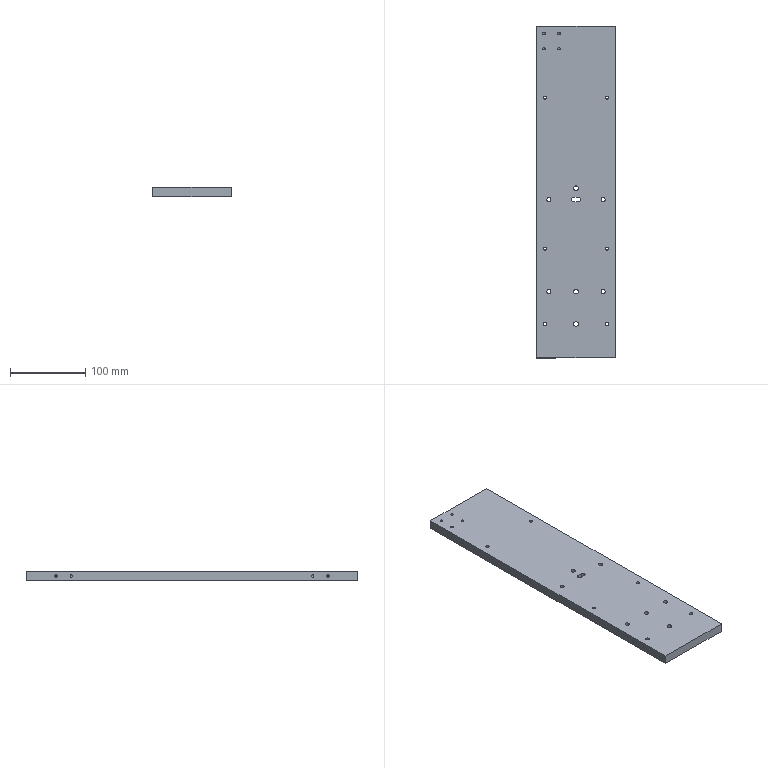Component | SolidWorks | 005-1 | 1 solid | 101 faces | box 105 x 440 x 12 mm | volume 548147 mm3 | cylinder 61 | cone 24 | plane 16 | commonest cylinder face diameters 3.3 x24 4.2 x12 6 x9 10 x8 5.5 x8 | material AL6061
build123d program:
from build123d import *

# Parameters (mm, degrees)
SKETCH1_W                                         = 105
SKETCH1_H                                         = 440
BOSS_EXTRUDE1_DEPTH                               = 12
CHAMFER1_SIZE                                     = 0.5
HOLE_SIZE_ACCORDING_TO_TYPE_OF_HEX_SO_D           = 5.5
HOLE_SIZE_ACCORDING_TO_TYPE_OF_HEX_SO_DEPTH       = 15
HOLE_SIZE_ACCORDING_TO_TYPE_OF_HEX_SO_CBORE_D     = 10
HOLE_SIZE_ACCORDING_TO_TYPE_OF_HEX_SO_CBORE_DEPTH = 5.7
HOLE_SIZE_ACCORDING_TO_TYPE_OF_HEX_SO_TIP         = 1.652
SKETCH4_R                                         = 3
CUT_EXTRUDE1_DEPTH                                = 227.496
M5_TAPPED_HOLE1_D                                 = 4.2
M5_TAPPED_HOLE1_DEPTH                             = 12.4
M5_TAPPED_HOLE1_TIP                               = 1.262
SIZE_MM_DOWEL_PIN_HOLE1_D                         = 6
SIZE_MM_DOWEL_PIN_HOLE1_DEPTH                     = 12.4
SIZE_MM_DOWEL_PIN_HOLE1_TIP                       = 1.803
M4_TAPPED_HOLE1_D                                 = 3.3
M4_TAPPED_HOLE1_DEPTH                             = 10.1
M4_TAPPED_HOLE1_TIP                               = 0.9914
M4_TAPPED_HOLE2_AT_2_COUNT                        = 2
M4_TAPPED_HOLE2_AT_2_PITCH                        = 20
M4_TAPPED_HOLE2_AT_3_COUNT                        = 2
M4_TAPPED_HOLE2_AT_3_PITCH                        = 360
M4_TAPPED_HOLE2_AT_4_COUNT                        = 2
M4_TAPPED_HOLE2_AT_4_PITCH                        = 340


with BuildPart() as part:
    # Sketch1 → Boss-Extrude1 (new body)
    with BuildSketch(Plane.XY):
        Rectangle(SKETCH1_W, SKETCH1_H)
    extrude(amount=BOSS_EXTRUDE1_DEPTH)

    # Chamfer1
    chamfer1_edges = [part.edges().sort_by_distance(p)[0] for p in [
        (52.5, -220, 6),
        (-52.5, -220, 6),
        (-52.5, 220, 6),
        (52.5, 220, 6),
    ]]
    chamfer(chamfer1_edges, length=CHAMFER1_SIZE)

    # Hole Size _ according to_ type of hex so
    with Locations(Plane.XY.offset(12)):
        with Locations((-36, -10), (36, -132), (-36, -132), (36, -10)):
            CounterBoreHole(HOLE_SIZE_ACCORDING_TO_TYPE_OF_HEX_SO_D / 2, HOLE_SIZE_ACCORDING_TO_TYPE_OF_HEX_SO_CBORE_D / 2, HOLE_SIZE_ACCORDING_TO_TYPE_OF_HEX_SO_CBORE_DEPTH, depth=HOLE_SIZE_ACCORDING_TO_TYPE_OF_HEX_SO_DEPTH)
            with Locations((0, 0, -(HOLE_SIZE_ACCORDING_TO_TYPE_OF_HEX_SO_DEPTH + HOLE_SIZE_ACCORDING_TO_TYPE_OF_HEX_SO_TIP / 2))):  # 118° drill point
                Cone(0, HOLE_SIZE_ACCORDING_TO_TYPE_OF_HEX_SO_D / 2, HOLE_SIZE_ACCORDING_TO_TYPE_OF_HEX_SO_TIP, mode=Mode.SUBTRACT)

    # Sketch4 → Cut-Extrude1 (cut, through all)
    with BuildSketch(Plane.XY.offset(12)):
        with Locations((0, -132)):
            Circle(SKETCH4_R)
        with BuildLine():
            Line((-3, -7), (3, -7))
            ThreePointArc((3, -7), (6, -10), (3, -13))
            Line((3, -13), (-3, -13))
            ThreePointArc((-3, -13), (-6, -10), (-3, -7))
        make_face()
    extrude(amount=-CUT_EXTRUDE1_DEPTH, mode=Mode.SUBTRACT)

    # M5 Tapped Hole1
    with Locations(Plane.XY.offset(12)):
        with Locations((-41, -175), (41, -75), (-41, -75), (41, -175), (41, 125), (-41, 125)):
            Hole(M5_TAPPED_HOLE1_D / 2, depth=M5_TAPPED_HOLE1_DEPTH)
            with Locations((0, 0, -(M5_TAPPED_HOLE1_DEPTH + M5_TAPPED_HOLE1_TIP / 2))):  # 118° drill point
                Cone(0, M5_TAPPED_HOLE1_D / 2, M5_TAPPED_HOLE1_TIP, mode=Mode.SUBTRACT)

    # Size mm Dowel Pin Hole1
    with Locations(Plane.XY.offset(12)):
        with Locations((0, -175), (0, 5)):
            Hole(SIZE_MM_DOWEL_PIN_HOLE1_D / 2, depth=SIZE_MM_DOWEL_PIN_HOLE1_DEPTH)
            with Locations((0, 0, -(SIZE_MM_DOWEL_PIN_HOLE1_DEPTH + SIZE_MM_DOWEL_PIN_HOLE1_TIP / 2))):  # 118° drill point
                Cone(0, SIZE_MM_DOWEL_PIN_HOLE1_D / 2, SIZE_MM_DOWEL_PIN_HOLE1_TIP, mode=Mode.SUBTRACT)

    # M4 Tapped Hole1
    with Locations(Plane(origin=(0, 0, 0), x_dir=(-1, 0, 0), z_dir=(0, 0, -1))):
        with Locations((-42.5, 210), (-22.5, 190), (-42.5, 190), (-22.5, 210)):
            Hole(M4_TAPPED_HOLE1_D / 2, depth=M4_TAPPED_HOLE1_DEPTH)
            with Locations((0, 0, -(M4_TAPPED_HOLE1_DEPTH + M4_TAPPED_HOLE1_TIP / 2))):  # 118° drill point
                Cone(0, M4_TAPPED_HOLE1_D / 2, M4_TAPPED_HOLE1_TIP, mode=Mode.SUBTRACT)

    # Sketch13 → M4 Tapped Hole2 (revolve, cut)
    with BuildSketch(Plane(origin=(-52.5, 180, 6), x_dir=(0, 0, 1), z_dir=(0, 1, 0))):
        Polygon((0, 0), (0, 11.091), (1.65, 10.1), (1.65, 0), align=None)
    m4_tapped_hole2 = revolve(axis=Axis((-58.85, 180, 6), (1, 0, 0)), mode=Mode.SUBTRACT)

    # M4 Tapped Hole2 at 2: M4 Tapped Hole2 ×2
    with Locations(*[(0, -i * M4_TAPPED_HOLE2_AT_2_PITCH, 0) for i in range(1, M4_TAPPED_HOLE2_AT_2_COUNT)]):
        add(m4_tapped_hole2, mode=Mode.SUBTRACT)

    # M4 Tapped Hole2 at 3: M4 Tapped Hole2 ×2
    with Locations(*[(0, -i * M4_TAPPED_HOLE2_AT_3_PITCH, 0) for i in range(1, M4_TAPPED_HOLE2_AT_3_COUNT)]):
        add(m4_tapped_hole2, mode=Mode.SUBTRACT)

    # M4 Tapped Hole2 at 4: M4 Tapped Hole2 ×2
    with Locations(*[(0, -i * M4_TAPPED_HOLE2_AT_4_PITCH, 0) for i in range(1, M4_TAPPED_HOLE2_AT_4_COUNT)]):
        add(m4_tapped_hole2, mode=Mode.SUBTRACT)

    # Mirror1: M4 Tapped Hole2 across plane
    add(m4_tapped_hole2.mirror(Plane.ZY), mode=Mode.SUBTRACT)

    # Mirror1 copy 1 sketch → Mirror1 copy 1 (revolve, cut)
    with BuildSketch(Plane(origin=(52.5, 160, 6), x_dir=(0, 0, 1), z_dir=(0, 1, 0))):
        Polygon((0, 0), (0, -11.091), (1.65, -10.1), (1.65, 0), align=None)
    revolve(axis=Axis((58.85, 160, 6), (1, 0, 0)), mode=Mode.SUBTRACT)

    # Mirror1 copy 2 sketch → Mirror1 copy 2 (revolve, cut)
    with BuildSketch(Plane(origin=(52.5, -180, 6), x_dir=(0, 0, 1), z_dir=(0, 1, 0))):
        Polygon((0, 0), (0, -11.091), (1.65, -10.1), (1.65, 0), align=None)
    revolve(axis=Axis((58.85, -180, 6), (1, 0, 0)), mode=Mode.SUBTRACT)

    # Mirror1 copy 3 sketch → Mirror1 copy 3 (revolve, cut)
    with BuildSketch(Plane(origin=(52.5, -160, 6), x_dir=(0, 0, 1), z_dir=(0, 1, 0))):
        Polygon((0, 0), (0, -11.091), (1.65, -10.1), (1.65, 0), align=None)
    revolve(axis=Axis((58.85, -160, 6), (1, 0, 0)), mode=Mode.SUBTRACT)


solid = part.part

# Placed as in the assembly
solid = solid.moved(Location((-238.955, -136.942, 166.696), (-180, 0, 180)))